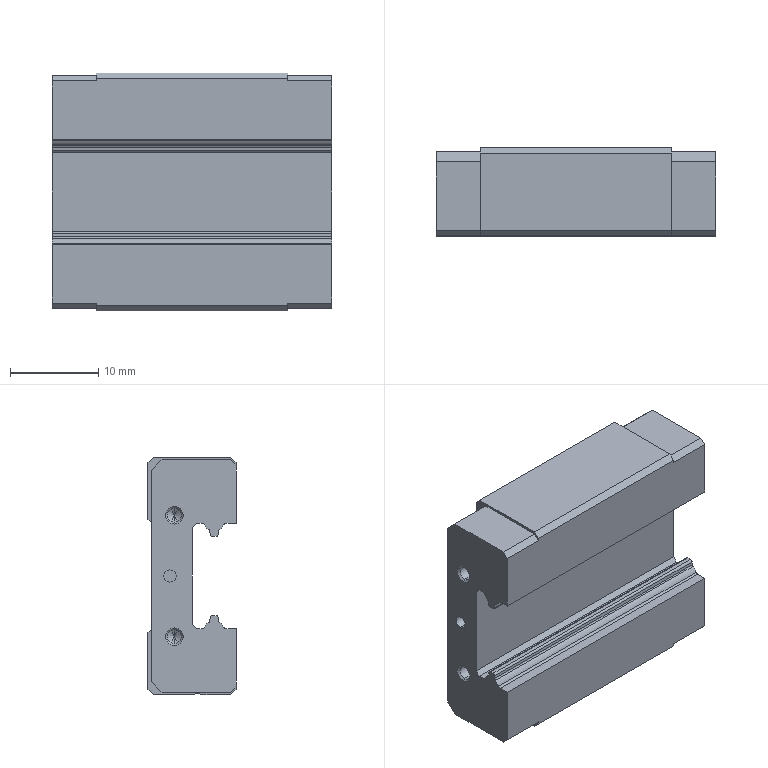Component | SolidWorks | 17268MGN12CZ0HM-1 | 1 solid | 116 faces | box 31.7 x 10 x 27 mm | volume 6337 mm3 | plane 47 | cylinder 37 | cone 32 | commonest cylinder face diameters 0.5 x12 1.567 x8 2.459 x8 1.4 x4 2.4 x4 1 x1 | material SKD-11 HRC58° Hard Chrome Plated
build123d program:
from build123d import *

# Parameters (mm, degrees)
BOSS_EXTRUDE1_DEPTH      = 10.85
BOSS_EXTRUDE1_DEPTH_BACK = 10.85
BOSS_EXTRUDE2_DEPTH      = 15.85
BOSS_EXTRUDE2_DEPTH_BACK = 15.85
CUT_EXTRUDE1_DEPTH       = 10.85
CUT_EXTRUDE1_DEPTH_BACK  = 10.85
CUT_EXTRUDE2_DEPTH       = 10.85
CUT_EXTRUDE2_DEPTH_BACK  = 10.85
CUT_EXTRUDE3_DEPTH       = 10.85
CUT_EXTRUDE3_DEPTH_BACK  = 10.85
CUT_EXTRUDE4_DEPTH       = 10.85
CUT_EXTRUDE4_DEPTH_BACK  = 10.85
SKETCH6_R                = 0.5
LPATTERN1_COUNT          = 2
LPATTERN1_PITCH          = 15
LPATTERN1_COUNT_DIR2     = 2
LPATTERN1_PITCH_DIR2     = 20
SKETCH9_W                = 5
SKETCH9_H                = 0.7
SKETCH14_W               = 5
SKETCH14_H               = 0.7


with BuildPart() as part:
    # Sketch1 → Boss-Extrude1 (new, two sides: drawn at the far end of the back side and taken through both)
    with BuildSketch(Plane(origin=(0, 0, 0), x_dir=(0, 0, -1), z_dir=(1, 0, 0)).offset(-BOSS_EXTRUDE1_DEPTH_BACK)):
        Polygon((-13.5, 0.6), (-12.9, 0), (12.9, 0), (13.5, 0.6), (13.5, 9.4), (12.9, 10), (6.4, 10), (6, 9.6), (-6, 9.6), (-6.4, 10), (-12.9, 10), (-13.5, 9.4), align=None)
    extrude(amount=BOSS_EXTRUDE1_DEPTH + BOSS_EXTRUDE1_DEPTH_BACK)

    # Sketch2 → Boss-Extrude2 (add, two sides: drawn at the far end of the back side and taken through both)
    with BuildSketch(Plane(origin=(0, 0, 0), x_dir=(0, 0, -1), z_dir=(1, 0, 0)).offset(-BOSS_EXTRUDE2_DEPTH_BACK)):
        Polygon((-13.2, 0.6), (-12.6, 0), (12.6, 0), (13.2, 0.6), (13.2, 8.4), (12, 9.6), (-12, 9.6), (-13.2, 8.4), align=None)
    extrude(amount=BOSS_EXTRUDE2_DEPTH + BOSS_EXTRUDE2_DEPTH_BACK)

    # Sketch3 → Cut-Extrude1 (cut, two sides: drawn at the far end of the back side and taken through both)
    with BuildSketch(Plane(origin=(0, 0, 0), x_dir=(0, 0, -1), z_dir=(1, 0, 0)).offset(-CUT_EXTRUDE1_DEPTH_BACK)):
        with BuildLine():
            Line((-6, -2.5), (-5.5, -3))
            Line((-5.5, -3), (1.6, -3))
            ThreePointArc((1.6, -3), (2, -2.8), (2.4, -3))
            Line((2.4, -3), (5.5, -3))
            Line((5.5, -3), (6, -2.5))
            Line((6, -2.5), (6, 1.142))
            ThreePointArc((6, 1.142), (5.956, 1.284), (5.838, 1.376))
            ThreePointArc((5.838, 1.376), (5.514, 1.576), (5.27, 1.868))
            ThreePointArc((5.27, 1.868), (5.187, 1.956), (5.074, 1.995))
            Line((5.074, 1.995), (4.728, 2.025))
            ThreePointArc((4.728, 2.025), (4.566, 2.105), (4.5, 2.274))
            Line((4.5, 2.274), (4.5, 2.694))
            ThreePointArc((4.5, 2.694), (4.566, 2.863), (4.728, 2.943))
            Line((4.728, 2.943), (5.074, 2.973))
            ThreePointArc((5.074, 2.973), (5.187, 3.012), (5.27, 3.1))
            ThreePointArc((5.27, 3.1), (5.514, 3.391), (5.838, 3.592))
            ThreePointArc((5.838, 3.592), (5.956, 3.683), (6, 3.825))
            Line((6, 3.825), (6, 4.5))
            Line((6, 4.5), (5.5, 5))
            Line((5.5, 5), (-5.5, 5))
            Line((-5.5, 5), (-6, 4.5))
            Line((-6, 4.5), (-6, 3.825))
            ThreePointArc((-6, 3.825), (-5.956, 3.683), (-5.838, 3.592))
            ThreePointArc((-5.838, 3.592), (-5.514, 3.391), (-5.27, 3.1))
            ThreePointArc((-5.27, 3.1), (-5.187, 3.012), (-5.074, 2.973))
            Line((-5.074, 2.973), (-4.728, 2.943))
            ThreePointArc((-4.728, 2.943), (-4.566, 2.863), (-4.5, 2.694))
            Line((-4.5, 2.694), (-4.5, 2.274))
            ThreePointArc((-4.5, 2.274), (-4.566, 2.105), (-4.728, 2.025))
            Line((-4.728, 2.025), (-5.074, 1.995))
            ThreePointArc((-5.074, 1.995), (-5.187, 1.956), (-5.27, 1.868))
            ThreePointArc((-5.27, 1.868), (-5.514, 1.576), (-5.838, 1.376))
            ThreePointArc((-5.838, 1.376), (-5.956, 1.284), (-6, 1.142))
            Line((-6, 1.142), (-6, -2.5))
        make_face()
    extrude(amount=CUT_EXTRUDE1_DEPTH + CUT_EXTRUDE1_DEPTH_BACK, mode=Mode.SUBTRACT)

    # Sketch4 → Cut-Extrude2 (cut, two sides: drawn at the far end of the back side and taken through both)
    with BuildSketch(Plane(origin=(10.85, 0, 0), x_dir=(0, 0, -1), z_dir=(1, 0, 0)).offset(-CUT_EXTRUDE2_DEPTH_BACK)):
        with BuildLine():
            Line((-6, -2.5), (-5.5, -3))
            Line((-5.5, -3), (1.6, -3))
            ThreePointArc((1.6, -3), (2, -2.8), (2.4, -3))
            Line((2.4, -3), (5.5, -3))
            Line((5.5, -3), (6, -2.5))
            Line((6, -2.5), (6, 1.142))
            ThreePointArc((6, 1.142), (5.956, 1.284), (5.838, 1.376))
            ThreePointArc((5.838, 1.376), (5.514, 1.576), (5.27, 1.868))
            ThreePointArc((5.27, 1.868), (5.187, 1.956), (5.074, 1.995))
            Line((5.074, 1.995), (4.728, 2.025))
            ThreePointArc((4.728, 2.025), (4.566, 2.105), (4.5, 2.274))
            Line((4.5, 2.274), (4.5, 2.694))
            ThreePointArc((4.5, 2.694), (4.566, 2.863), (4.728, 2.943))
            Line((4.728, 2.943), (5.074, 2.973))
            ThreePointArc((5.074, 2.973), (5.187, 3.012), (5.27, 3.1))
            ThreePointArc((5.27, 3.1), (5.514, 3.391), (5.838, 3.592))
            ThreePointArc((5.838, 3.592), (5.956, 3.683), (6, 3.825))
            Line((6, 3.825), (6, 4.5))
            Line((6, 4.5), (5.5, 5))
            Line((5.5, 5), (-5.5, 5))
            Line((-5.5, 5), (-6, 4.5))
            Line((-6, 4.5), (-6, 3.825))
            ThreePointArc((-6, 3.825), (-5.956, 3.683), (-5.838, 3.592))
            ThreePointArc((-5.838, 3.592), (-5.514, 3.391), (-5.27, 3.1))
            ThreePointArc((-5.27, 3.1), (-5.187, 3.012), (-5.074, 2.973))
            Line((-5.074, 2.973), (-4.728, 2.943))
            ThreePointArc((-4.728, 2.943), (-4.566, 2.863), (-4.5, 2.694))
            Line((-4.5, 2.694), (-4.5, 2.274))
            ThreePointArc((-4.5, 2.274), (-4.566, 2.105), (-4.728, 2.025))
            Line((-4.728, 2.025), (-5.074, 1.995))
            ThreePointArc((-5.074, 1.995), (-5.187, 1.956), (-5.27, 1.868))
            ThreePointArc((-5.27, 1.868), (-5.514, 1.576), (-5.838, 1.376))
            ThreePointArc((-5.838, 1.376), (-5.956, 1.284), (-6, 1.142))
            Line((-6, 1.142), (-6, -2.5))
        make_face()
    extrude(amount=CUT_EXTRUDE2_DEPTH + CUT_EXTRUDE2_DEPTH_BACK, mode=Mode.SUBTRACT)

    # Sketch5 → Cut-Extrude3 (cut, two sides: drawn at the far end of the back side and taken through both)
    with BuildSketch(Plane(origin=(-10.85, 0, 0), x_dir=(0, 0, -1), z_dir=(1, 0, 0)).offset(-CUT_EXTRUDE3_DEPTH_BACK)):
        with BuildLine():
            Line((-6, -2.5), (-5.5, -3))
            Line((-5.5, -3), (1.6, -3))
            ThreePointArc((1.6, -3), (2, -2.8), (2.4, -3))
            Line((2.4, -3), (5.5, -3))
            Line((5.5, -3), (6, -2.5))
            Line((6, -2.5), (6, 1.142))
            ThreePointArc((6, 1.142), (5.956, 1.284), (5.838, 1.376))
            ThreePointArc((5.838, 1.376), (5.514, 1.576), (5.27, 1.868))
            ThreePointArc((5.27, 1.868), (5.187, 1.956), (5.074, 1.995))
            Line((5.074, 1.995), (4.728, 2.025))
            ThreePointArc((4.728, 2.025), (4.566, 2.105), (4.5, 2.274))
            Line((4.5, 2.274), (4.5, 2.694))
            ThreePointArc((4.5, 2.694), (4.566, 2.863), (4.728, 2.943))
            Line((4.728, 2.943), (5.074, 2.973))
            ThreePointArc((5.074, 2.973), (5.187, 3.012), (5.27, 3.1))
            ThreePointArc((5.27, 3.1), (5.514, 3.391), (5.838, 3.592))
            ThreePointArc((5.838, 3.592), (5.956, 3.683), (6, 3.825))
            Line((6, 3.825), (6, 4.5))
            Line((6, 4.5), (5.5, 5))
            Line((5.5, 5), (-5.5, 5))
            Line((-5.5, 5), (-6, 4.5))
            Line((-6, 4.5), (-6, 3.825))
            ThreePointArc((-6, 3.825), (-5.956, 3.683), (-5.838, 3.592))
            ThreePointArc((-5.838, 3.592), (-5.514, 3.391), (-5.27, 3.1))
            ThreePointArc((-5.27, 3.1), (-5.187, 3.012), (-5.074, 2.973))
            Line((-5.074, 2.973), (-4.728, 2.943))
            ThreePointArc((-4.728, 2.943), (-4.566, 2.863), (-4.5, 2.694))
            Line((-4.5, 2.694), (-4.5, 2.274))
            ThreePointArc((-4.5, 2.274), (-4.566, 2.105), (-4.728, 2.025))
            Line((-4.728, 2.025), (-5.074, 1.995))
            ThreePointArc((-5.074, 1.995), (-5.187, 1.956), (-5.27, 1.868))
            ThreePointArc((-5.27, 1.868), (-5.514, 1.576), (-5.838, 1.376))
            ThreePointArc((-5.838, 1.376), (-5.956, 1.284), (-6, 1.142))
            Line((-6, 1.142), (-6, -2.5))
        make_face()
    extrude(amount=CUT_EXTRUDE3_DEPTH + CUT_EXTRUDE3_DEPTH_BACK, mode=Mode.SUBTRACT)

    # Sketch6 → Cut-Extrude4 (cut, two sides: drawn at the far end of the back side and taken through both)
    with BuildSketch(Plane(origin=(0, 0, 0), x_dir=(0, 0, -1), z_dir=(1, 0, 0)).offset(-CUT_EXTRUDE4_DEPTH_BACK)):
        with Locations((13.8, 4.4)):
            Circle(SKETCH6_R)
    extrude(amount=CUT_EXTRUDE4_DEPTH + CUT_EXTRUDE4_DEPTH_BACK, mode=Mode.SUBTRACT)

    # Sketch7 → Cut-Revolve1 (revolve, cut)
    with BuildSketch(Plane.XY.offset(-10), mode=Mode.PRIVATE) as cut_revolve1_sk:
        Polygon((7.5, 4.39), (6.271, 5.1), (6.271, 9.729), (6, 10), (7.5, 10), align=None)
    cut_revolve1 = revolve(cut_revolve1_sk.sketch.rotate(Axis((7.5, 10, -10), (0, -1, 0)), 270), axis=Axis((7.5, 10, -10), (0, -1, 0)), mode=Mode.SUBTRACT)

    # LPattern1: Cut-Revolve1 2 × 2
    with Locations(*[(-i * LPATTERN1_PITCH, 0, j * LPATTERN1_PITCH_DIR2) for i in range(LPATTERN1_COUNT) for j in range(LPATTERN1_COUNT_DIR2) if (i, j) != (0, 0)]):
        add(cut_revolve1, mode=Mode.SUBTRACT)

    # Sketch9 → Cut-Revolve2 (revolve, cut)
    with BuildSketch(Plane.XY, mode=Mode.PRIVATE) as cut_revolve2_sk:
        with Locations((-13.35, 7.85)):
            Rectangle(SKETCH9_W, SKETCH9_H)
    revolve(cut_revolve2_sk.sketch.rotate(Axis((-10.85, 7.5, 0), (-1, 0, 0)), 270), axis=Axis((-10.85, 7.5, 0), (-1, 0, 0)), mode=Mode.SUBTRACT)

    # Sketch10 → Cut-Revolve3 (revolve, cut)
    with BuildSketch(Plane.XY.offset(6.9), mode=Mode.PRIVATE) as cut_revolve3_sk:
        Polygon((-15.85, 7), (-15.85, 8), (-15.633, 7.784), (-10.85, 7.784), (-10.398, 7), align=None)
    revolve(cut_revolve3_sk.sketch.rotate(Axis((-10.398, 7, 6.9), (-1, 0, 0)), 270), axis=Axis((-10.398, 7, 6.9), (-1, 0, 0)), mode=Mode.SUBTRACT)

    # Sketch11 → Cut-Revolve4 (revolve, cut)
    with BuildSketch(Plane.XY.offset(6.9), mode=Mode.PRIVATE) as cut_revolve4_sk:
        Polygon((10.398, 7), (10.85, 7.784), (15.633, 7.784), (15.85, 8), (15.85, 7), align=None)
    revolve(cut_revolve4_sk.sketch.rotate(Axis((15.85, 7, 6.9), (-1, 0, 0)), 270), axis=Axis((15.85, 7, 6.9), (-1, 0, 0)), mode=Mode.SUBTRACT)

    # Sketch12 → Cut-Revolve5 (revolve, cut)
    with BuildSketch(Plane.XY.offset(-6.9), mode=Mode.PRIVATE) as cut_revolve5_sk:
        Polygon((-15.85, 7), (-15.85, 8), (-15.633, 7.784), (-10.85, 7.784), (-10.398, 7), align=None)
    revolve(cut_revolve5_sk.sketch.rotate(Axis((-10.398, 7, -6.9), (-1, 0, 0)), 270), axis=Axis((-10.398, 7, -6.9), (-1, 0, 0)), mode=Mode.SUBTRACT)

    # Sketch13 → Cut-Revolve6 (revolve, cut)
    with BuildSketch(Plane.XY.offset(-6.9), mode=Mode.PRIVATE) as cut_revolve6_sk:
        Polygon((10.398, 7), (10.85, 7.784), (15.633, 7.784), (15.85, 8), (15.85, 7), align=None)
    revolve(cut_revolve6_sk.sketch.rotate(Axis((15.85, 7, -6.9), (-1, 0, 0)), 270), axis=Axis((15.85, 7, -6.9), (-1, 0, 0)), mode=Mode.SUBTRACT)

    # Sketch14 → Cut-Revolve7 (revolve, cut)
    with BuildSketch(Plane.XY, mode=Mode.PRIVATE) as cut_revolve7_sk:
        with Locations((13.35, 7.85)):
            Rectangle(SKETCH14_W, SKETCH14_H)
    revolve(cut_revolve7_sk.sketch.rotate(Axis((15.85, 7.5, 0), (-1, 0, 0)), 270), axis=Axis((15.85, 7.5, 0), (-1, 0, 0)), mode=Mode.SUBTRACT)


solid = part.part

# Placed as in the assembly
solid = solid.moved(Location((22.65, -40.579, 0), (0, 0, 0)))